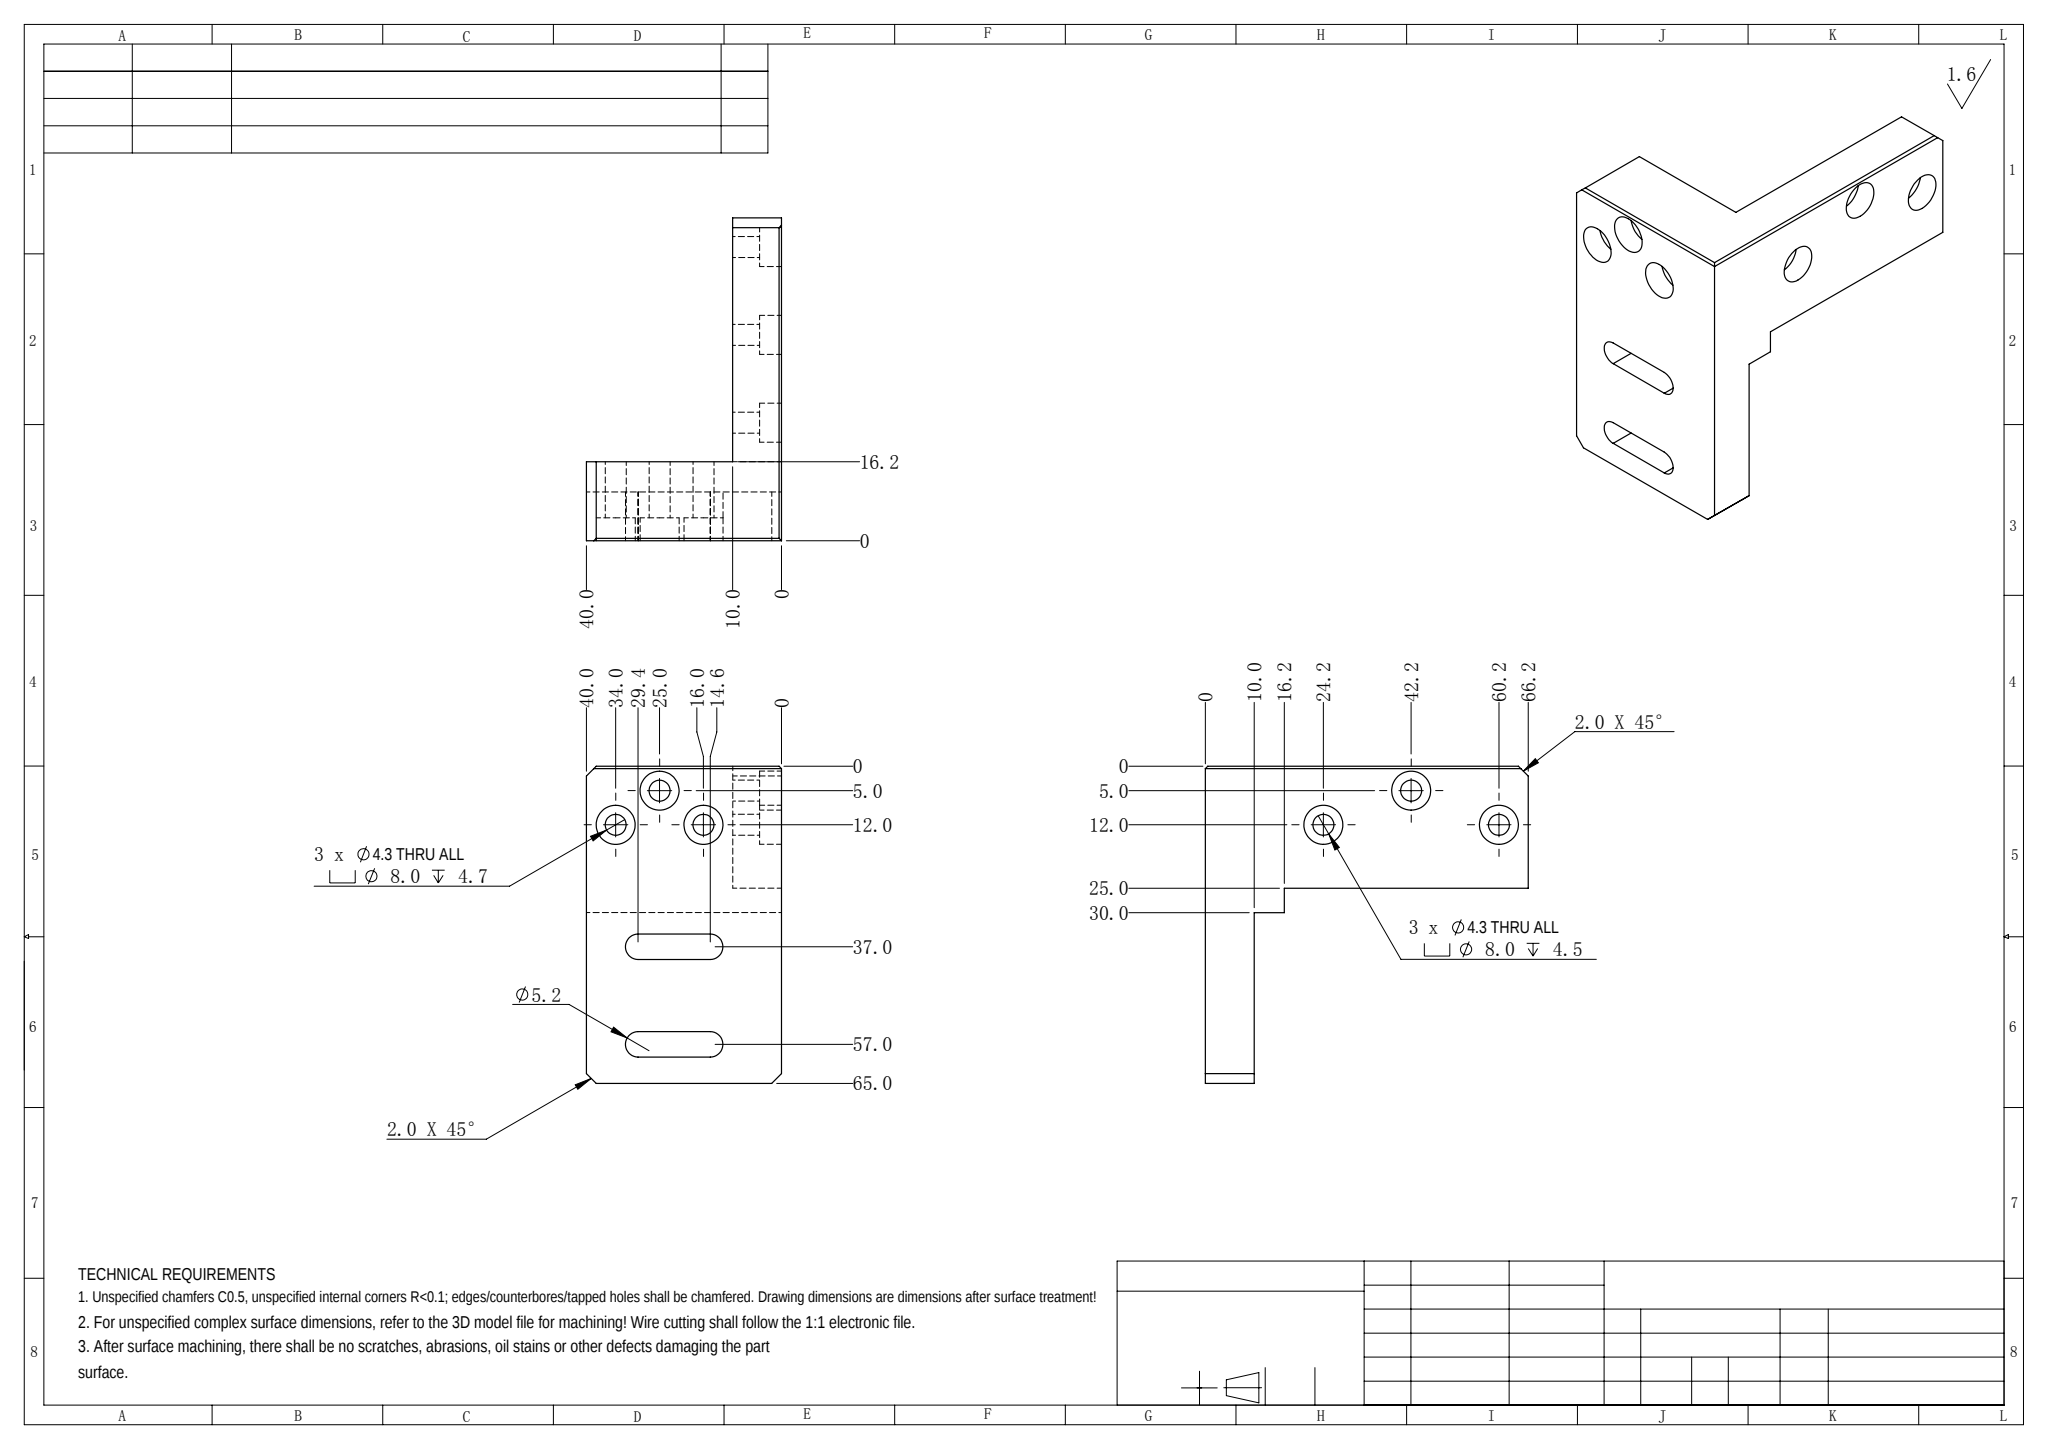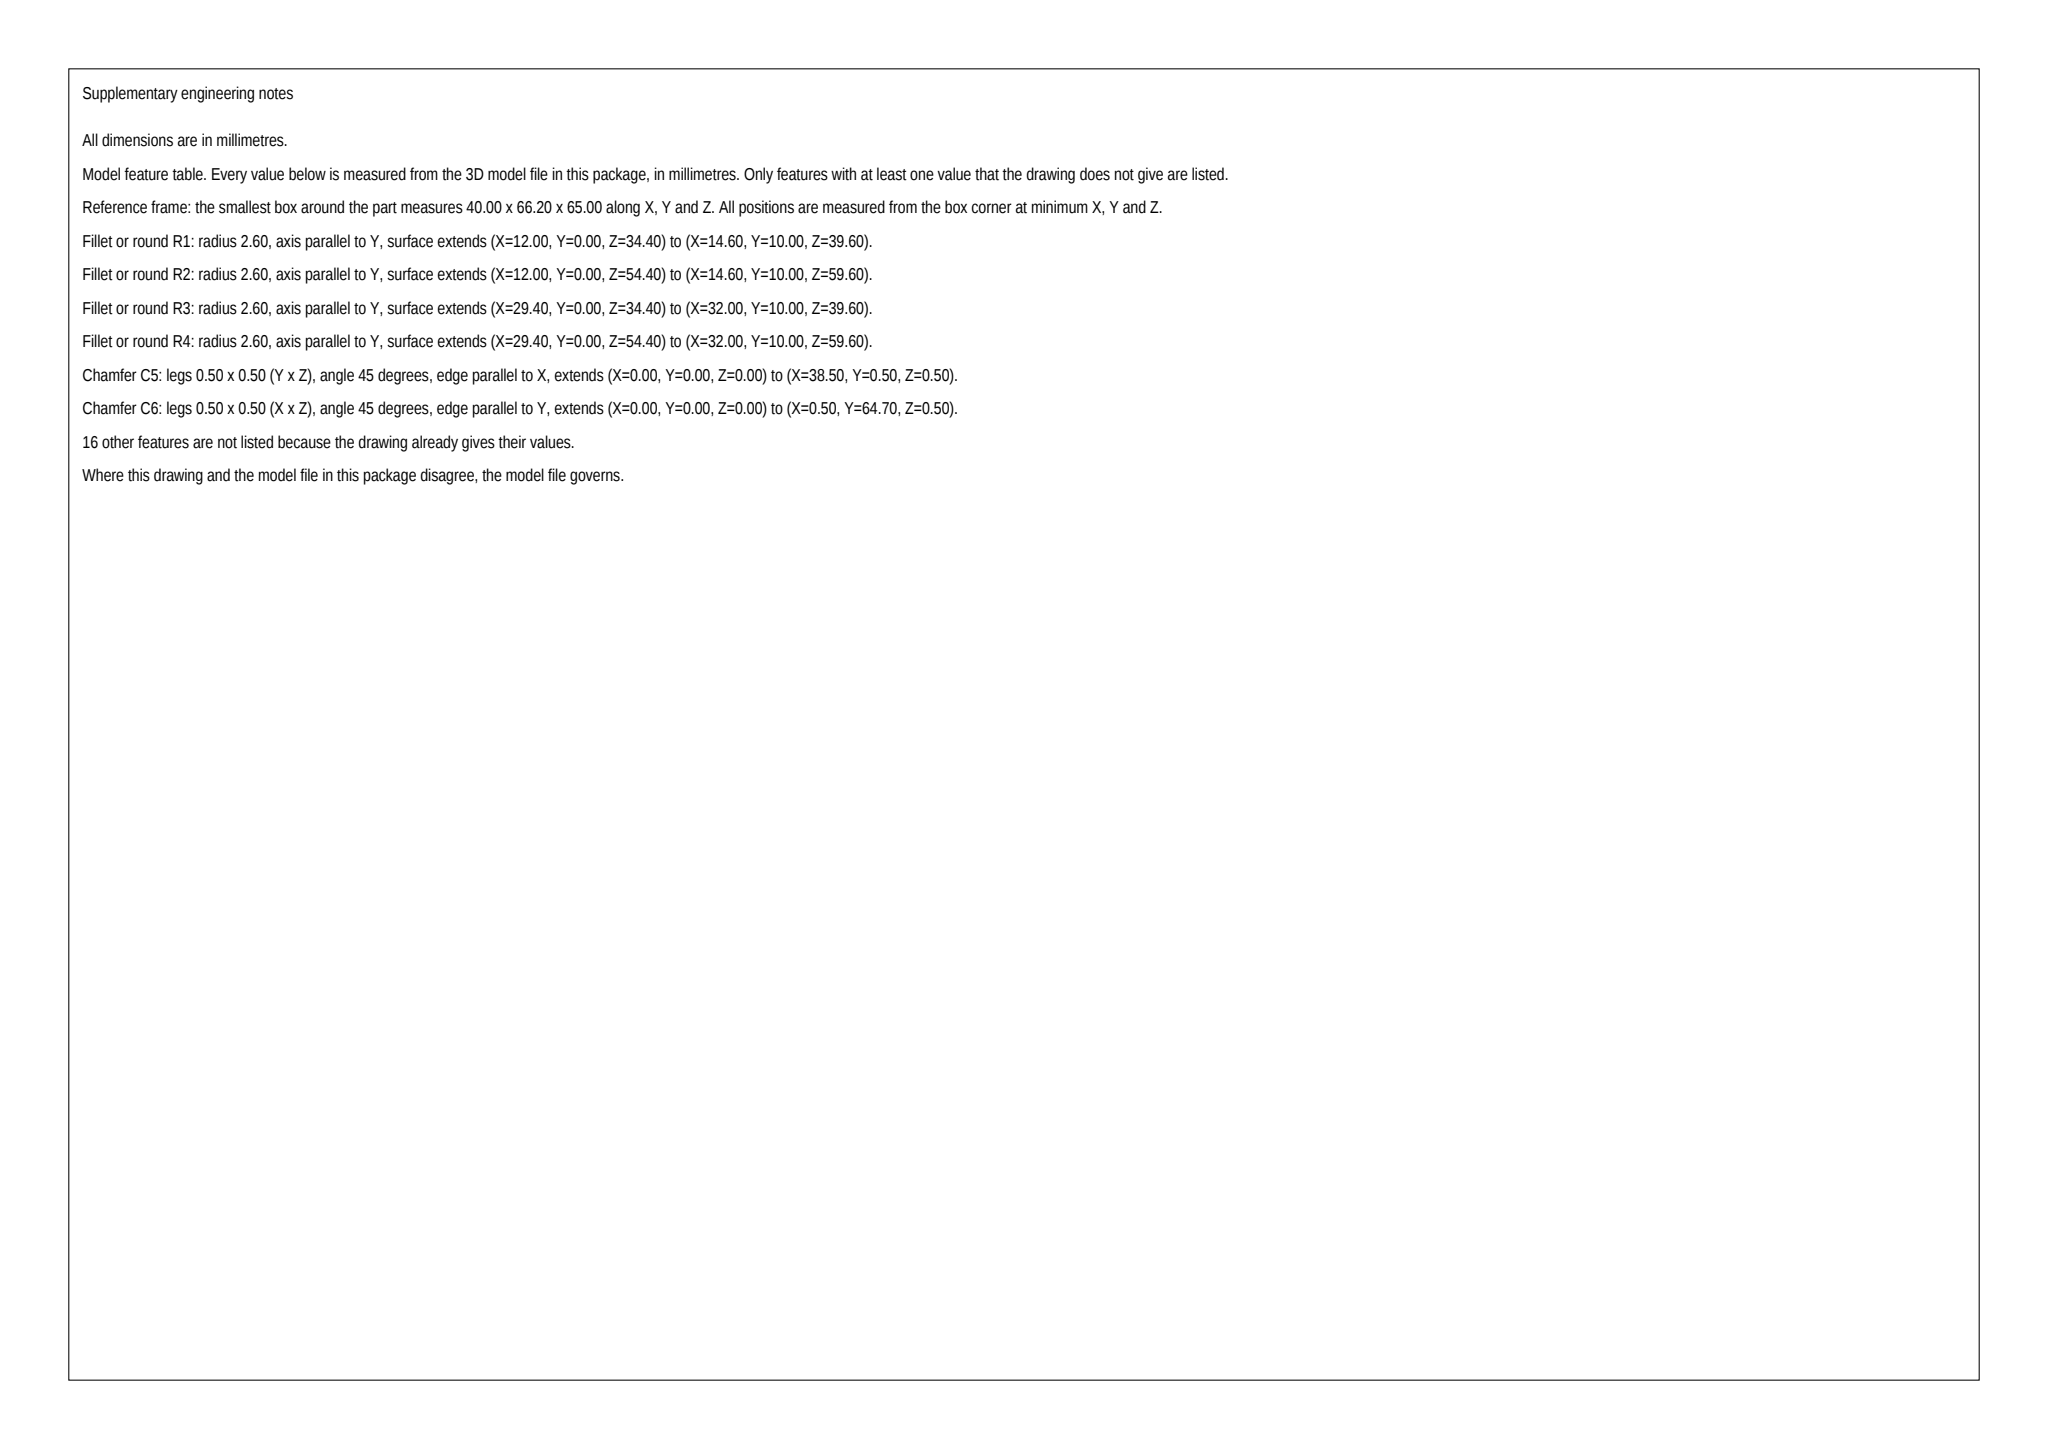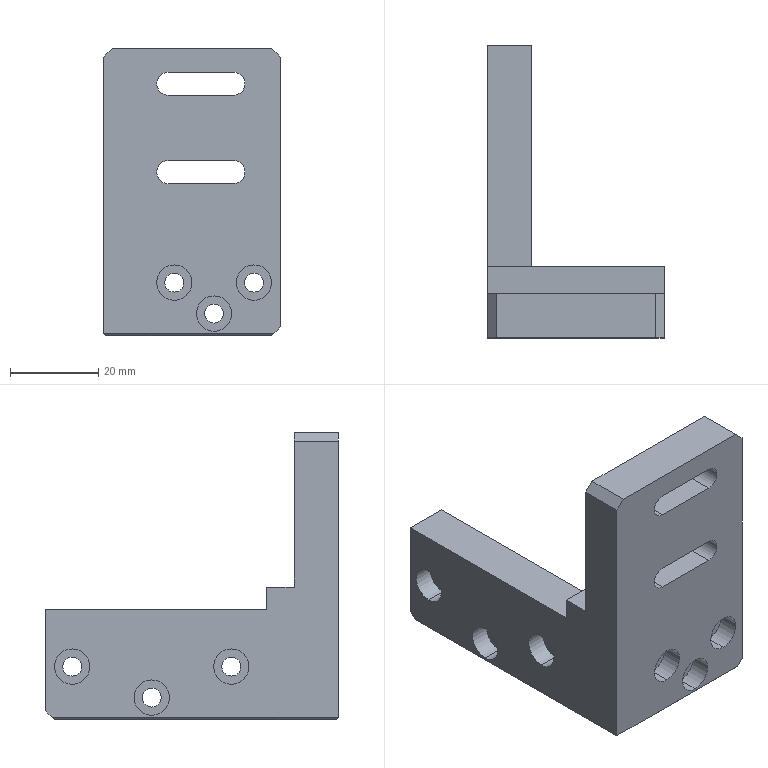Part | SolidWorks | mm | 1 solid | 55 faces | box 40 x 66.2 x 65 mm | volume 41743 mm3 | cylinder 28 | plane 27 | commonest cylinder face diameters 8 x12 4.3 x12 5.2 x4